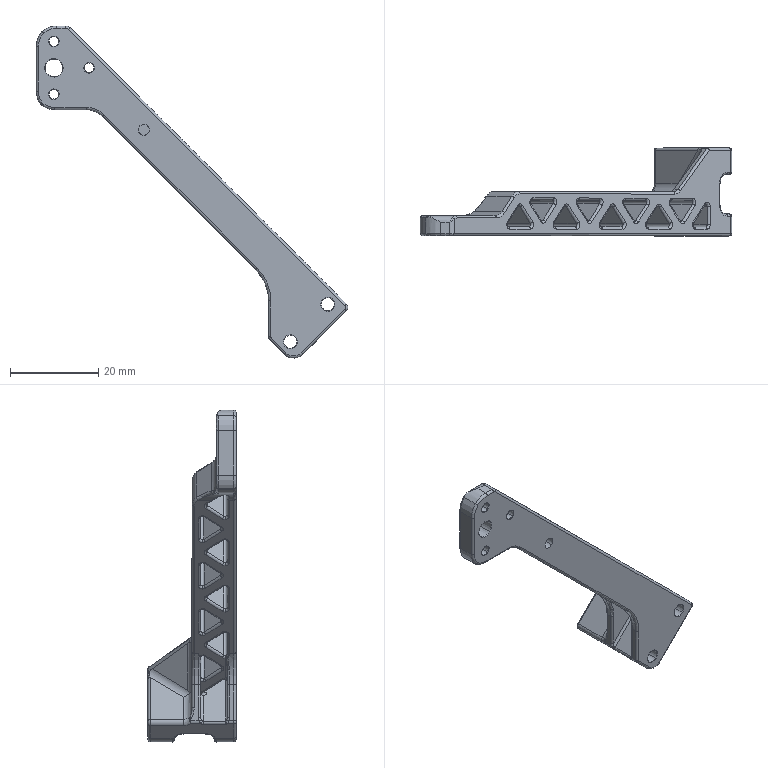Component | SolidWorks | 3.Spider arm-1 | 1 solid | 378 faces | box 70.76 x 20 x 75.43 mm | volume 7575 mm3 | cylinder 164 | torus 127 | plane 50 | spline 33 | sphere 4 | commonest cylinder face diameters 1 x122 4 x8 2.2 x6 3 x6 2 x5 10 x5 6 x4 0.2 x4